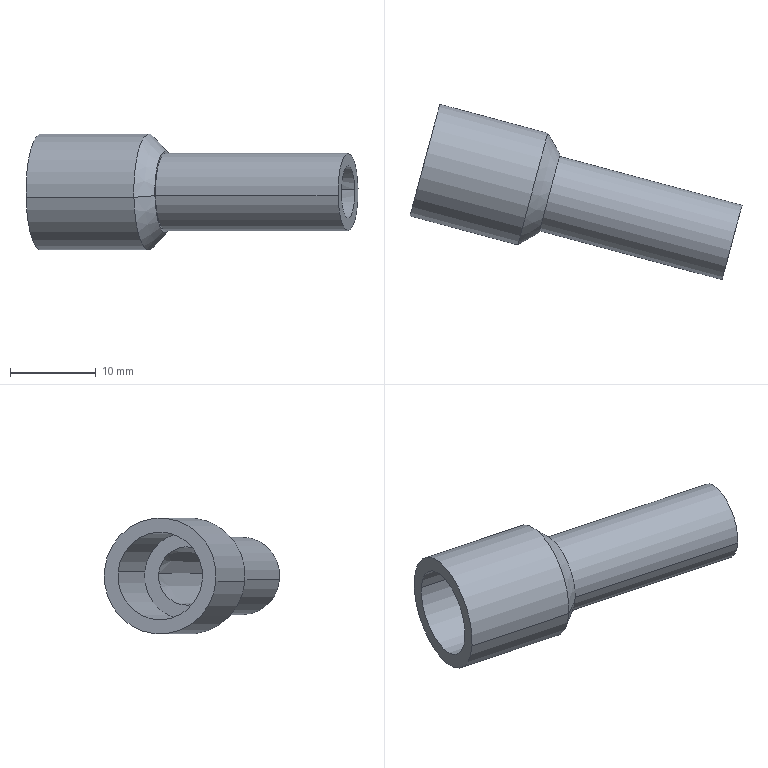Component | SolidWorks | ScrewFeedConnectorAssembly-1_ScrewFeedConnector-1 | 1 solid | 14 faces | box 38.65 x 20.44 x 13.5 mm | volume 1672 mm3 | cylinder 6 | cone 4 | plane 4 | commonest cylinder face diameters 10.2 x2 13.5 x2 9 x2
build123d program:
from build123d import *

# Parameters (mm, degrees)
BOSS_EXTRUDE1_START = 12
SKETCH2_R           = 6.75
SKETCH2_R_2         = 5.1
BOSS_EXTRUDE1_DEPTH = 12
CHAMFER1_SIZE       = 2


with BuildPart() as part:
    # Sketch1 → Revolve1 (revolve)
    with BuildSketch(Plane.XY, mode=Mode.PRIVATE) as revolve1_sk:
        Polygon((3.05, 0), (4.5, 0), (4.5, 22), (6.75, 22), (6.75, 25), (3.4, 25), align=None)
    revolve(revolve1_sk.sketch.rotate(Axis((0, -1.55, 0), (0, 1, 0)), 90), axis=Axis((0, -1.55, 0), (0, 1, 0)))

    # Sketch2 → Boss-Extrude1 (add)
    with BuildSketch(Plane(origin=(0, 25, 0), x_dir=(1, 0, 0), z_dir=(0, 1, 0)).offset(BOSS_EXTRUDE1_START)):
        with Locations(Location((0, 0, 0), (0, 0, 90))):
            Circle(SKETCH2_R)
        with Locations(Location((0, 0, 0), (0, 0, 270))):
            Circle(SKETCH2_R_2, mode=Mode.SUBTRACT)
    extrude(amount=-BOSS_EXTRUDE1_DEPTH)

    # Chamfer1
    chamfer1_edges = [part.edges().sort_by_distance(p)[0] for p in [
        (0, 22, 6.75),
    ]]
    chamfer(chamfer1_edges, length=CHAMFER1_SIZE)


solid = part.part

# Placed as in the assembly
solid = solid.moved(Location((16.411, 84.726, 11), (93.992, -14.965, 91.032)))
STEP:
#1=COLOUR_RGB('',0.7922,0.8196,0.9333);
#2=FILL_AREA_STYLE_COLOUR('',#1);
#3=FILL_AREA_STYLE('',(#2));
#4=SURFACE_STYLE_FILL_AREA(#3);
#5=SURFACE_SIDE_STYLE('',(#4));
#6=SURFACE_STYLE_USAGE(.BOTH.,#5);
#7=PRESENTATION_STYLE_ASSIGNMENT((#6));
#8=CARTESIAN_POINT('',(-0.1423,3.74,0.4503));
#9=VERTEX_POINT('',#8);
#10=CARTESIAN_POINT('',(-0.2387,3.38,0.4158));
#11=VERTEX_POINT('',#10);
#12=CARTESIAN_POINT('',(-0.1905,3.56,0.4331));
#13=DIRECTION('',(0.9659,-0.2588,0.));
#14=DIRECTION('',(0.2577,0.9618,0.09214));
#15=AXIS2_PLACEMENT_3D('',#12,#13,#14);
#16=CIRCLE('',#15,0.187);
#17=EDGE_CURVE('',#9,#11,#16,.T.);
#18=ORIENTED_EDGE('',*,*,#17,.F.);
#19=CARTESIAN_POINT('',(-0.1981,3.836,0.4576));
#20=VERTEX_POINT('',#19);
#21=CARTESIAN_POINT('',(-0.1423,3.74,0.4503));
#22=DIRECTION('',(-0.5008,0.8631,0.06515));
#23=VECTOR('',#22,39.37);
#24=LINE('',#21,#23);
#25=EDGE_CURVE('',#9,#20,#24,.T.);
#26=ORIENTED_EDGE('',*,*,#25,.T.);
#27=CARTESIAN_POINT('',(-0.3351,3.325,0.4086));
#28=VERTEX_POINT('',#27);
#29=CARTESIAN_POINT('',(-0.2666,3.58,0.4331));
#30=DIRECTION('',(-0.9659,0.2588,-0.));
#31=DIRECTION('',(0.2577,0.9618,0.09214));
#32=AXIS2_PLACEMENT_3D('',#29,#30,#31);
#33=CIRCLE('',#32,0.2657);
#34=EDGE_CURVE('',#28,#20,#33,.T.);
#35=ORIENTED_EDGE('',*,*,#34,.F.);
#36=CARTESIAN_POINT('',(-0.2387,3.38,0.4158));
#37=DIRECTION('',(-0.8652,-0.4971,-0.06515));
#38=VECTOR('',#37,39.37);
#39=LINE('',#36,#38);
#40=EDGE_CURVE('',#11,#28,#39,.T.);
#41=ORIENTED_EDGE('',*,*,#40,.F.);
#42=EDGE_LOOP('',(#18,#26,#35,#41));
#43=FACE_OUTER_BOUND('',#42,.T.);
#44=CARTESIAN_POINT('',(-0.1905,3.56,0.4331));
#45=DIRECTION('',(-0.9659,0.2588,-0.));
#46=DIRECTION('',(-0.2577,-0.9618,-0.09214));
#47=AXIS2_PLACEMENT_3D('',#44,#45,#46);
#48=CONICAL_SURFACE('',#47,0.187,0.7854);
#49=ADVANCED_FACE('',(#43),#48,.T.);
#50=CARTESIAN_POINT('',(-0.7092,3.906,0.4516));
#51=VERTEX_POINT('',#50);
#52=CARTESIAN_POINT('',(-0.8127,3.52,0.4146));
#53=VERTEX_POINT('',#52);
#54=CARTESIAN_POINT('',(-0.7609,3.713,0.4331));
#55=DIRECTION('',(-0.9659,0.2588,-0.));
#56=DIRECTION('',(-0.2577,-0.9618,-0.09214));
#57=AXIS2_PLACEMENT_3D('',#54,#55,#56);
#58=CIRCLE('',#57,0.2008);
#59=EDGE_CURVE('',#51,#53,#58,.T.);
#60=ORIENTED_EDGE('',*,*,#59,.T.);
#61=CARTESIAN_POINT('',(-0.3563,3.397,0.4146));
#62=VERTEX_POINT('',#61);
#63=CARTESIAN_POINT('',(-0.8127,3.52,0.4146));
#64=DIRECTION('',(0.9659,-0.2588,0.));
#65=VECTOR('',#64,39.37);
#66=LINE('',#63,#65);
#67=EDGE_CURVE('',#53,#62,#66,.T.);
#68=ORIENTED_EDGE('',*,*,#67,.T.);
#69=CARTESIAN_POINT('',(-0.2529,3.784,0.4516));
#70=VERTEX_POINT('',#69);
#71=CARTESIAN_POINT('',(-0.3046,3.59,0.4331));
#72=DIRECTION('',(0.9659,-0.2588,0.));
#73=DIRECTION('',(-0.2577,-0.9618,-0.09214));
#74=AXIS2_PLACEMENT_3D('',#71,#72,#73);
#75=CIRCLE('',#74,0.2008);
#76=EDGE_CURVE('',#62,#70,#75,.T.);
#77=ORIENTED_EDGE('',*,*,#76,.T.);
#78=CARTESIAN_POINT('',(-0.7092,3.906,0.4516));
#79=DIRECTION('',(0.9659,-0.2588,0.));
#80=VECTOR('',#79,39.37);
#81=LINE('',#78,#80);
#82=EDGE_CURVE('',#51,#70,#81,.T.);
#83=ORIENTED_EDGE('',*,*,#82,.F.);
#84=EDGE_LOOP('',(#60,#68,#77,#83));
#85=FACE_OUTER_BOUND('',#84,.T.);
#86=CARTESIAN_POINT('',(-0.7609,3.713,0.4331));
#87=DIRECTION('',(0.9659,-0.2588,0.));
#88=DIRECTION('',(0.2577,0.9618,0.09214));
#89=AXIS2_PLACEMENT_3D('',#86,#87,#88);
#90=CYLINDRICAL_SURFACE('',#89,0.2008);
#91=ADVANCED_FACE('',(#85),#90,.F.);
#92=CARTESIAN_POINT('',(-0.8294,3.457,0.4086));
#93=VERTEX_POINT('',#92);
#94=CARTESIAN_POINT('',(-0.6925,3.968,0.4576));
#95=VERTEX_POINT('',#94);
#96=CARTESIAN_POINT('',(-0.7609,3.713,0.4331));
#97=DIRECTION('',(-0.9659,0.2588,-0.));
#98=DIRECTION('',(-0.2577,-0.9618,-0.09214));
#99=AXIS2_PLACEMENT_3D('',#96,#97,#98);
#100=CIRCLE('',#99,0.2657);
#101=EDGE_CURVE('',#93,#95,#100,.T.);
#102=ORIENTED_EDGE('',*,*,#101,.F.);
#103=CARTESIAN_POINT('',(0.6366,3.064,0.4086));
#104=DIRECTION('',(0.9659,-0.2588,0.));
#105=VECTOR('',#104,39.37);
#106=LINE('',#103,#105);
#107=EDGE_CURVE('',#93,#28,#106,.T.);
#108=ORIENTED_EDGE('',*,*,#107,.T.);
#109=ORIENTED_EDGE('',*,*,#34,.T.);
#110=CARTESIAN_POINT('',(0.7736,3.575,0.4576));
#111=DIRECTION('',(0.9659,-0.2588,0.));
#112=VECTOR('',#111,39.37);
#113=LINE('',#110,#112);
#114=EDGE_CURVE('',#95,#20,#113,.T.);
#115=ORIENTED_EDGE('',*,*,#114,.F.);
#116=EDGE_LOOP('',(#102,#108,#109,#115));
#117=FACE_OUTER_BOUND('',#116,.T.);
#118=CARTESIAN_POINT('',(0.7051,3.32,0.4331));
#119=DIRECTION('',(0.9659,-0.2588,0.));
#120=DIRECTION('',(0.2577,0.9618,0.09214));
#121=AXIS2_PLACEMENT_3D('',#118,#119,#120);
#122=CYLINDRICAL_SURFACE('',#121,0.2657);
#123=ADVANCED_FACE('',(#117),#122,.T.);
#124=CARTESIAN_POINT('',(0.6152,3.22,0.422));
#125=VERTEX_POINT('',#124);
#126=CARTESIAN_POINT('',(0.6771,3.451,0.4441));
#127=VERTEX_POINT('',#126);
#128=CARTESIAN_POINT('',(0.6461,3.336,0.4331));
#129=DIRECTION('',(0.9659,-0.2588,0.));
#130=DIRECTION('',(0.2577,0.9618,0.09214));
#131=AXIS2_PLACEMENT_3D('',#128,#129,#130);
#132=CIRCLE('',#131,0.1201);
#133=EDGE_CURVE('',#125,#127,#132,.T.);
#134=ORIENTED_EDGE('',*,*,#133,.T.);
#135=CARTESIAN_POINT('',(-0.2701,3.719,0.4454));
#136=VERTEX_POINT('',#135);
#137=CARTESIAN_POINT('',(-0.2701,3.719,0.4454));
#138=DIRECTION('',(-0.9622,0.2723,0.00129));
#139=VECTOR('',#138,39.37);
#140=LINE('',#137,#139);
#141=EDGE_CURVE('',#127,#136,#140,.T.);
#142=ORIENTED_EDGE('',*,*,#141,.T.);
#143=CARTESIAN_POINT('',(-0.3391,3.462,0.4207));
#144=VERTEX_POINT('',#143);
#145=CARTESIAN_POINT('',(-0.3046,3.59,0.4331));
#146=DIRECTION('',(0.9659,-0.2588,0.));
#147=DIRECTION('',(0.2577,0.9618,0.09214));
#148=AXIS2_PLACEMENT_3D('',#145,#146,#147);
#149=CIRCLE('',#148,0.1339);
#150=EDGE_CURVE('',#144,#136,#149,.T.);
#151=ORIENTED_EDGE('',*,*,#150,.F.);
#152=CARTESIAN_POINT('',(-0.3391,3.462,0.4207));
#153=DIRECTION('',(-0.9694,0.2453,-0.00129));
#154=VECTOR('',#153,39.37);
#155=LINE('',#152,#154);
#156=EDGE_CURVE('',#125,#144,#155,.T.);
#157=ORIENTED_EDGE('',*,*,#156,.F.);
#158=EDGE_LOOP('',(#134,#142,#151,#157));
#159=FACE_OUTER_BOUND('',#158,.T.);
#160=CARTESIAN_POINT('',(-0.3046,3.59,0.4331));
#161=DIRECTION('',(-0.9659,0.2588,-0.));
#162=DIRECTION('',(-0.2577,-0.9618,-0.09214));
#163=AXIS2_PLACEMENT_3D('',#160,#161,#162);
#164=CONICAL_SURFACE('',#163,0.1339,0.014);
#165=ADVANCED_FACE('',(#159),#164,.F.);
#166=CARTESIAN_POINT('',(-0.1449,3.73,0.4494));
#167=VERTEX_POINT('',#166);
#168=CARTESIAN_POINT('',(-0.2362,3.389,0.4167));
#169=VERTEX_POINT('',#168);
#170=CARTESIAN_POINT('',(-0.1905,3.56,0.4331));
#171=DIRECTION('',(0.9659,-0.2588,0.));
#172=DIRECTION('',(0.2577,0.9618,0.09214));
#173=AXIS2_PLACEMENT_3D('',#170,#171,#172);
#174=CIRCLE('',#173,0.1772);
#175=EDGE_CURVE('',#167,#169,#174,.T.);
#176=ORIENTED_EDGE('',*,*,#175,.T.);
#177=CARTESIAN_POINT('',(0.6005,3.165,0.4167));
#178=VERTEX_POINT('',#177);
#179=CARTESIAN_POINT('',(0.6594,3.149,0.4167));
#180=DIRECTION('',(0.9659,-0.2588,0.));
#181=VECTOR('',#180,39.37);
#182=LINE('',#179,#181);
#183=EDGE_CURVE('',#169,#178,#182,.T.);
#184=ORIENTED_EDGE('',*,*,#183,.T.);
#185=CARTESIAN_POINT('',(0.6918,3.506,0.4494));
#186=VERTEX_POINT('',#185);
#187=CARTESIAN_POINT('',(0.6461,3.336,0.4331));
#188=DIRECTION('',(0.9659,-0.2588,0.));
#189=DIRECTION('',(0.2577,0.9618,0.09214));
#190=AXIS2_PLACEMENT_3D('',#187,#188,#189);
#191=CIRCLE('',#190,0.1772);
#192=EDGE_CURVE('',#186,#178,#191,.T.);
#193=ORIENTED_EDGE('',*,*,#192,.F.);
#194=CARTESIAN_POINT('',(0.7507,3.49,0.4494));
#195=DIRECTION('',(0.9659,-0.2588,0.));
#196=VECTOR('',#195,39.37);
#197=LINE('',#194,#196);
#198=EDGE_CURVE('',#167,#186,#197,.T.);
#199=ORIENTED_EDGE('',*,*,#198,.F.);
#200=EDGE_LOOP('',(#176,#184,#193,#199));
#201=FACE_OUTER_BOUND('',#200,.T.);
#202=CARTESIAN_POINT('',(0.7051,3.32,0.4331));
#203=DIRECTION('',(0.9659,-0.2588,0.));
#204=DIRECTION('',(0.2577,0.9618,0.09214));
#205=AXIS2_PLACEMENT_3D('',#202,#203,#204);
#206=CYLINDRICAL_SURFACE('',#205,0.1772);
#207=ADVANCED_FACE('',(#201),#206,.T.);
#208=ORIENTED_EDGE('',*,*,#183,.F.);
#209=CARTESIAN_POINT('',(-0.1905,3.56,0.4331));
#210=DIRECTION('',(0.9659,-0.2588,0.));
#211=DIRECTION('',(0.2577,0.9618,0.09214));
#212=AXIS2_PLACEMENT_3D('',#209,#210,#211);
#213=CIRCLE('',#212,0.1772);
#214=EDGE_CURVE('',#169,#167,#213,.T.);
#215=ORIENTED_EDGE('',*,*,#214,.T.);
#216=ORIENTED_EDGE('',*,*,#198,.T.);
#217=CARTESIAN_POINT('',(0.6461,3.336,0.4331));
#218=DIRECTION('',(0.9659,-0.2588,0.));
#219=DIRECTION('',(0.2577,0.9618,0.09214));
#220=AXIS2_PLACEMENT_3D('',#217,#218,#219);
#221=CIRCLE('',#220,0.1772);
#222=EDGE_CURVE('',#178,#186,#221,.T.);
#223=ORIENTED_EDGE('',*,*,#222,.F.);
#224=EDGE_LOOP('',(#208,#215,#216,#223));
#225=FACE_OUTER_BOUND('',#224,.T.);
#226=CARTESIAN_POINT('',(0.7051,3.32,0.4331));
#227=DIRECTION('',(0.9659,-0.2588,0.));
#228=DIRECTION('',(0.2577,0.9618,0.09214));
#229=AXIS2_PLACEMENT_3D('',#226,#227,#228);
#230=CYLINDRICAL_SURFACE('',#229,0.1772);
#231=ADVANCED_FACE('',(#225),#230,.T.);
#232=ORIENTED_EDGE('',*,*,#192,.T.);
#233=ORIENTED_EDGE('',*,*,#222,.T.);
#234=EDGE_LOOP('',(#232,#233));
#235=FACE_OUTER_BOUND('',#234,.T.);
#236=ORIENTED_EDGE('',*,*,#133,.F.);
#237=CARTESIAN_POINT('',(0.6461,3.336,0.4331));
#238=DIRECTION('',(0.9659,-0.2588,0.));
#239=DIRECTION('',(0.2577,0.9618,0.09214));
#240=AXIS2_PLACEMENT_3D('',#237,#238,#239);
#241=CIRCLE('',#240,0.1201);
#242=EDGE_CURVE('',#127,#125,#241,.T.);
#243=ORIENTED_EDGE('',*,*,#242,.F.);
#244=EDGE_LOOP('',(#236,#243));
#245=FACE_BOUND('',#244,.T.);
#246=CARTESIAN_POINT('',(0.6433,3.325,0.5526));
#247=DIRECTION('',(0.9659,-0.2588,0.));
#248=DIRECTION('',(0.2577,0.9618,0.09214));
#249=AXIS2_PLACEMENT_3D('',#246,#247,#248);
#250=PLANE('',#249);
#251=ADVANCED_FACE('',(#235,#245),#250,.T.);
#252=ORIENTED_EDGE('',*,*,#141,.F.);
#253=ORIENTED_EDGE('',*,*,#242,.T.);
#254=ORIENTED_EDGE('',*,*,#156,.T.);
#255=CARTESIAN_POINT('',(-0.3046,3.59,0.4331));
#256=DIRECTION('',(0.9659,-0.2588,0.));
#257=DIRECTION('',(0.2577,0.9618,0.09214));
#258=AXIS2_PLACEMENT_3D('',#255,#256,#257);
#259=CIRCLE('',#258,0.1339);
#260=EDGE_CURVE('',#136,#144,#259,.T.);
#261=ORIENTED_EDGE('',*,*,#260,.F.);
#262=EDGE_LOOP('',(#252,#253,#254,#261));
#263=FACE_OUTER_BOUND('',#262,.T.);
#264=CARTESIAN_POINT('',(-0.3046,3.59,0.4331));
#265=DIRECTION('',(-0.9659,0.2588,-0.));
#266=DIRECTION('',(-0.2577,-0.9618,-0.09214));
#267=AXIS2_PLACEMENT_3D('',#264,#265,#266);
#268=CONICAL_SURFACE('',#267,0.1339,0.014);
#269=ADVANCED_FACE('',(#263),#268,.F.);
#270=CARTESIAN_POINT('',(-0.3046,3.59,0.4331));
#271=DIRECTION('',(0.9659,-0.2588,0.));
#272=DIRECTION('',(-0.2577,-0.9618,-0.09214));
#273=AXIS2_PLACEMENT_3D('',#270,#271,#272);
#274=CIRCLE('',#273,0.2008);
#275=EDGE_CURVE('',#70,#62,#274,.T.);
#276=ORIENTED_EDGE('',*,*,#275,.F.);
#277=ORIENTED_EDGE('',*,*,#76,.F.);
#278=EDGE_LOOP('',(#276,#277));
#279=FACE_OUTER_BOUND('',#278,.T.);
#280=ORIENTED_EDGE('',*,*,#150,.T.);
#281=ORIENTED_EDGE('',*,*,#260,.T.);
#282=EDGE_LOOP('',(#280,#281));
#283=FACE_BOUND('',#282,.T.);
#284=CARTESIAN_POINT('',(-0.3109,3.567,0.6977));
#285=DIRECTION('',(-0.9659,0.2588,-0.));
#286=DIRECTION('',(-0.2577,-0.9618,-0.09214));
#287=AXIS2_PLACEMENT_3D('',#284,#285,#286);
#288=PLANE('',#287);
#289=ADVANCED_FACE('',(#279,#283),#288,.T.);
#290=ORIENTED_EDGE('',*,*,#107,.F.);
#291=CARTESIAN_POINT('',(-0.7609,3.713,0.4331));
#292=DIRECTION('',(-0.9659,0.2588,-0.));
#293=DIRECTION('',(-0.2577,-0.9618,-0.09214));
#294=AXIS2_PLACEMENT_3D('',#291,#292,#293);
#295=CIRCLE('',#294,0.2657);
#296=EDGE_CURVE('',#95,#93,#295,.T.);
#297=ORIENTED_EDGE('',*,*,#296,.F.);
#298=ORIENTED_EDGE('',*,*,#114,.T.);
#299=CARTESIAN_POINT('',(-0.2666,3.58,0.4331));
#300=DIRECTION('',(-0.9659,0.2588,-0.));
#301=DIRECTION('',(0.2577,0.9618,0.09214));
#302=AXIS2_PLACEMENT_3D('',#299,#300,#301);
#303=CIRCLE('',#302,0.2657);
#304=EDGE_CURVE('',#20,#28,#303,.T.);
#305=ORIENTED_EDGE('',*,*,#304,.T.);
#306=EDGE_LOOP('',(#290,#297,#298,#305));
#307=FACE_OUTER_BOUND('',#306,.T.);
#308=CARTESIAN_POINT('',(0.7051,3.32,0.4331));
#309=DIRECTION('',(0.9659,-0.2588,0.));
#310=DIRECTION('',(0.2577,0.9618,0.09214));
#311=AXIS2_PLACEMENT_3D('',#308,#309,#310);
#312=CYLINDRICAL_SURFACE('',#311,0.2657);
#313=ADVANCED_FACE('',(#307),#312,.T.);
#314=CARTESIAN_POINT('',(-0.1905,3.56,0.4331));
#315=DIRECTION('',(0.9659,-0.2588,0.));
#316=DIRECTION('',(0.2577,0.9618,0.09214));
#317=AXIS2_PLACEMENT_3D('',#314,#315,#316);
#318=CIRCLE('',#317,0.187);
#319=EDGE_CURVE('',#11,#9,#318,.T.);
#320=ORIENTED_EDGE('',*,*,#319,.T.);
#321=ORIENTED_EDGE('',*,*,#17,.T.);
#322=EDGE_LOOP('',(#320,#321));
#323=FACE_OUTER_BOUND('',#322,.T.);
#324=ORIENTED_EDGE('',*,*,#175,.F.);
#325=ORIENTED_EDGE('',*,*,#214,.F.);
#326=EDGE_LOOP('',(#324,#325));
#327=FACE_BOUND('',#326,.T.);
#328=CARTESIAN_POINT('',(-0.1947,3.544,0.6095));
#329=DIRECTION('',(0.9659,-0.2588,0.));
#330=DIRECTION('',(0.2577,0.9618,0.09214));
#331=AXIS2_PLACEMENT_3D('',#328,#329,#330);
#332=PLANE('',#331);
#333=ADVANCED_FACE('',(#323,#327),#332,.T.);
#334=ORIENTED_EDGE('',*,*,#296,.T.);
#335=ORIENTED_EDGE('',*,*,#101,.T.);
#336=EDGE_LOOP('',(#334,#335));
#337=FACE_OUTER_BOUND('',#336,.T.);
#338=ORIENTED_EDGE('',*,*,#59,.F.);
#339=CARTESIAN_POINT('',(-0.7609,3.713,0.4331));
#340=DIRECTION('',(-0.9659,0.2588,-0.));
#341=DIRECTION('',(-0.2577,-0.9618,-0.09214));
#342=AXIS2_PLACEMENT_3D('',#339,#340,#341);
#343=CIRCLE('',#342,0.2008);
#344=EDGE_CURVE('',#53,#51,#343,.T.);
#345=ORIENTED_EDGE('',*,*,#344,.F.);
#346=EDGE_LOOP('',(#338,#345));
#347=FACE_BOUND('',#346,.T.);
#348=CARTESIAN_POINT('',(-0.7609,3.713,0.4331));
#349=DIRECTION('',(-0.9659,0.2588,-0.));
#350=DIRECTION('',(-0.2577,-0.9618,-0.09214));
#351=AXIS2_PLACEMENT_3D('',#348,#349,#350);
#352=PLANE('',#351);
#353=ADVANCED_FACE('',(#337,#347),#352,.T.);
#354=ORIENTED_EDGE('',*,*,#67,.F.);
#355=ORIENTED_EDGE('',*,*,#344,.T.);
#356=ORIENTED_EDGE('',*,*,#82,.T.);
#357=ORIENTED_EDGE('',*,*,#275,.T.);
#358=EDGE_LOOP('',(#354,#355,#356,#357));
#359=FACE_OUTER_BOUND('',#358,.T.);
#360=CARTESIAN_POINT('',(-0.7609,3.713,0.4331));
#361=DIRECTION('',(0.9659,-0.2588,0.));
#362=DIRECTION('',(0.2577,0.9618,0.09214));
#363=AXIS2_PLACEMENT_3D('',#360,#361,#362);
#364=CYLINDRICAL_SURFACE('',#363,0.2008);
#365=ADVANCED_FACE('',(#359),#364,.F.);
#366=ORIENTED_EDGE('',*,*,#25,.F.);
#367=ORIENTED_EDGE('',*,*,#319,.F.);
#368=ORIENTED_EDGE('',*,*,#40,.T.);
#369=ORIENTED_EDGE('',*,*,#304,.F.);
#370=EDGE_LOOP('',(#366,#367,#368,#369));
#371=FACE_OUTER_BOUND('',#370,.T.);
#372=CARTESIAN_POINT('',(-0.1905,3.56,0.4331));
#373=DIRECTION('',(-0.9659,0.2588,-0.));
#374=DIRECTION('',(-0.2577,-0.9618,-0.09214));
#375=AXIS2_PLACEMENT_3D('',#372,#373,#374);
#376=CONICAL_SURFACE('',#375,0.187,0.7854);
#377=ADVANCED_FACE('',(#371),#376,.T.);
#378=CLOSED_SHELL('',(#49,#91,#123,#165,#207,#231,#251,#269,#289,#313,#333,#353,#365,#377));
#379=MANIFOLD_SOLID_BREP('',#378);
#380=STYLED_ITEM('',(#7),#379);
#381=(LENGTH_UNIT()NAMED_UNIT(*)SI_UNIT($,.METRE.));
#382=LENGTH_MEASURE_WITH_UNIT(LENGTH_MEASURE(0.0254),#381);
#383=DIMENSIONAL_EXPONENTS(1.,0.,0.,0.,0.,0.,0.);
#384=(CONVERSION_BASED_UNIT('',#382)LENGTH_UNIT()NAMED_UNIT(#383));
#385=UNCERTAINTY_MEASURE_WITH_UNIT(LENGTH_MEASURE(0.00001),#384,'','');
#386=(NAMED_UNIT(*)PLANE_ANGLE_UNIT()SI_UNIT($,.RADIAN.));
#387=(NAMED_UNIT(*)SI_UNIT($,.STERADIAN.)SOLID_ANGLE_UNIT());
#388=(GEOMETRIC_REPRESENTATION_CONTEXT(3)GLOBAL_UNCERTAINTY_ASSIGNED_CONTEXT((#385))GLOBAL_UNIT_ASSIGNED_CONTEXT((#384,#386,#387))REPRESENTATION_CONTEXT('',''));
#389=MECHANICAL_DESIGN_GEOMETRIC_PRESENTATION_REPRESENTATION('',(#380),#388);
#390=CARTESIAN_POINT('',(0.,0.,0.));
#391=DIRECTION('',(0.,0.,1.));
#392=DIRECTION('',(1.,0.,0.));
#393=AXIS2_PLACEMENT_3D('',#390,#391,#392);
#394=(LENGTH_UNIT()NAMED_UNIT(*)SI_UNIT($,.METRE.));
#395=LENGTH_MEASURE_WITH_UNIT(LENGTH_MEASURE(0.0254),#394);
#396=DIMENSIONAL_EXPONENTS(1.,0.,0.,0.,0.,0.,0.);
#397=(CONVERSION_BASED_UNIT('',#395)LENGTH_UNIT()NAMED_UNIT(#396));
#398=UNCERTAINTY_MEASURE_WITH_UNIT(LENGTH_MEASURE(0.00001),#397,'','');
#399=(NAMED_UNIT(*)PLANE_ANGLE_UNIT()SI_UNIT($,.RADIAN.));
#400=(NAMED_UNIT(*)SI_UNIT($,.STERADIAN.)SOLID_ANGLE_UNIT());
#401=(GEOMETRIC_REPRESENTATION_CONTEXT(3)GLOBAL_UNCERTAINTY_ASSIGNED_CONTEXT((#398))GLOBAL_UNIT_ASSIGNED_CONTEXT((#397,#399,#400))REPRESENTATION_CONTEXT('',''));
#402=ADVANCED_BREP_SHAPE_REPRESENTATION('',(#379,#393),#401);
#403=PRESENTATION_LAYER_ASSIGNMENT('','',(#380));